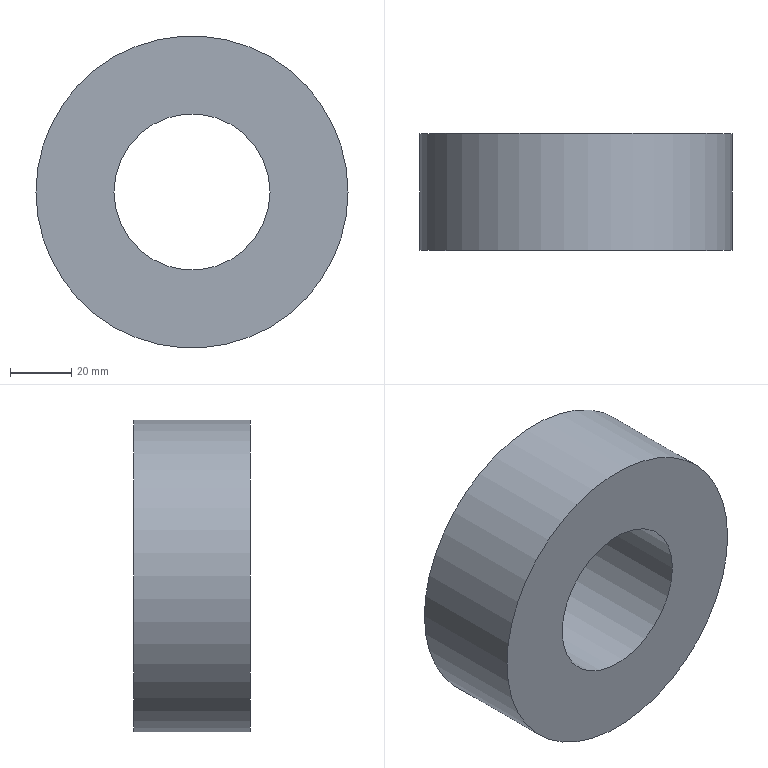Component | NX | WASHER_2 | 1 solid | 4 faces | volume 231059 mm3 | cylinder 2 | plane 2 | commonest cylinder face diameters 101.6 x1 50.8 x1